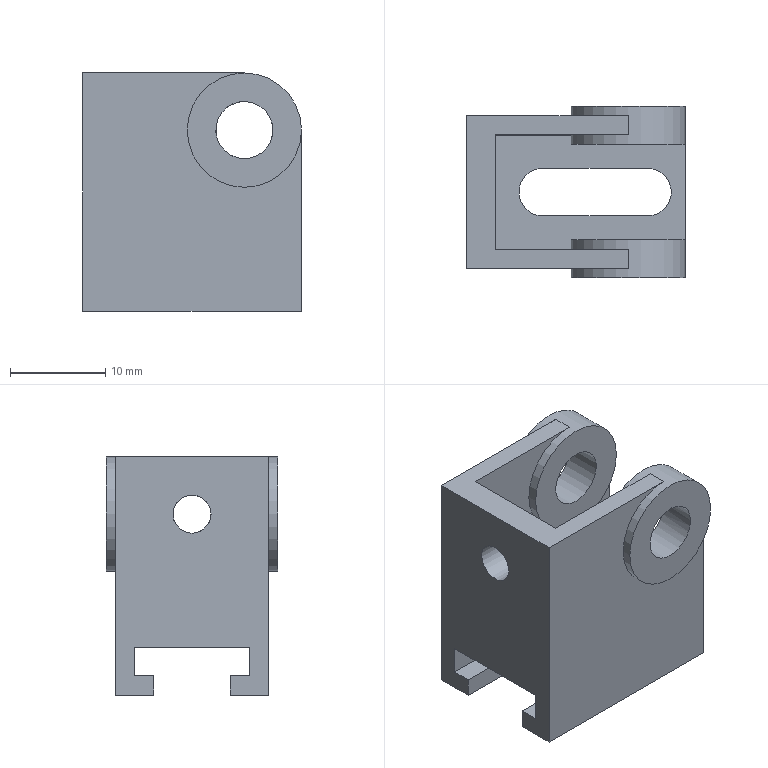Component | NX | LINK_SLIDER | 1 solid | 31 faces | volume 3858 mm3 | plane 24 | cylinder 7 | commonest cylinder face diameters 12 x2 6 x2 5 x2 4 x1